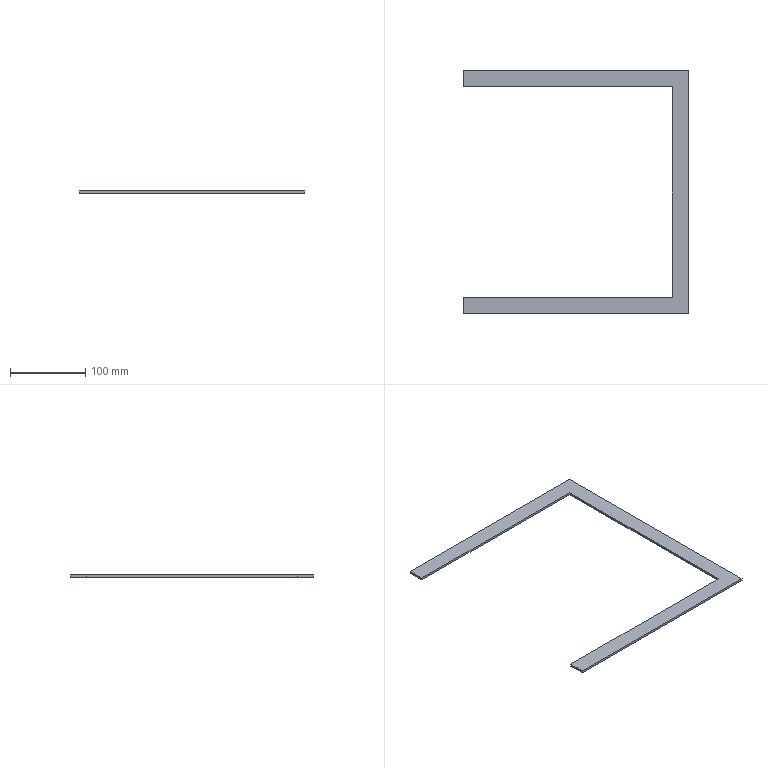Component | SolidWorks | Cover1-9XG1-1 | 1 solid | 10 faces | box 300 x 324 x 3 mm | volume 58080 mm3 | plane 10
build123d program:
from build123d import *

# Parameters (mm, degrees)
BOSS_EXTRUDE1_DEPTH = 3


with BuildPart() as part:
    # Sketch1 → Boss-Extrude1 (new body)
    with BuildSketch(Plane.XY):
        Polygon((-162, 0), (162, 0), (162, 300), (140, 300), (140, 22), (-140, 22), (-140, 300), (-162, 300), align=None)
    extrude(amount=BOSS_EXTRUDE1_DEPTH)


solid = part.part

# Placed as in the assembly
solid = solid.moved(Location((150, 0, -3), (0, 0, 90)))
STEP:
#1=CARTESIAN_POINT('',(-5.906,-6.378,-0.1181));
#2=VERTEX_POINT('',#1);
#3=CARTESIAN_POINT('',(5.906,-6.378,-0.1181));
#4=VERTEX_POINT('',#3);
#5=CARTESIAN_POINT('',(-5.906,-6.378,-0.1181));
#6=DIRECTION('',(1.,0.,-0.));
#7=VECTOR('',#6,39.37);
#8=LINE('',#5,#7);
#9=EDGE_CURVE('',#2,#4,#8,.T.);
#10=ORIENTED_EDGE('',*,*,#9,.T.);
#11=CARTESIAN_POINT('',(5.906,-6.378,-0.));
#12=VERTEX_POINT('',#11);
#13=CARTESIAN_POINT('',(5.906,-6.378,-0.));
#14=DIRECTION('',(0.,-0.,-1.));
#15=VECTOR('',#14,39.37);
#16=LINE('',#13,#15);
#17=EDGE_CURVE('',#12,#4,#16,.T.);
#18=ORIENTED_EDGE('',*,*,#17,.F.);
#19=CARTESIAN_POINT('',(-5.906,-6.378,-0.));
#20=VERTEX_POINT('',#19);
#21=CARTESIAN_POINT('',(-5.906,-6.378,-0.));
#22=DIRECTION('',(1.,0.,-0.));
#23=VECTOR('',#22,39.37);
#24=LINE('',#21,#23);
#25=EDGE_CURVE('',#20,#12,#24,.T.);
#26=ORIENTED_EDGE('',*,*,#25,.F.);
#27=CARTESIAN_POINT('',(-5.906,-6.378,-0.));
#28=DIRECTION('',(0.,-0.,-1.));
#29=VECTOR('',#28,39.37);
#30=LINE('',#27,#29);
#31=EDGE_CURVE('',#20,#2,#30,.T.);
#32=ORIENTED_EDGE('',*,*,#31,.T.);
#33=EDGE_LOOP('',(#10,#18,#26,#32));
#34=FACE_OUTER_BOUND('',#33,.T.);
#35=CARTESIAN_POINT('',(-5.906,-6.378,-0.));
#36=DIRECTION('',(-0.,1.,-0.));
#37=DIRECTION('',(-1.,-0.,0.));
#38=AXIS2_PLACEMENT_3D('',#35,#36,#37);
#39=PLANE('',#38);
#40=ADVANCED_FACE('',(#34),#39,.F.);
#41=CARTESIAN_POINT('',(5.906,6.378,-0.1181));
#42=VERTEX_POINT('',#41);
#43=CARTESIAN_POINT('',(5.906,-6.378,-0.1181));
#44=DIRECTION('',(0.,1.,-0.));
#45=VECTOR('',#44,39.37);
#46=LINE('',#43,#45);
#47=EDGE_CURVE('',#4,#42,#46,.T.);
#48=ORIENTED_EDGE('',*,*,#47,.T.);
#49=CARTESIAN_POINT('',(5.906,6.378,-0.));
#50=VERTEX_POINT('',#49);
#51=CARTESIAN_POINT('',(5.906,6.378,-0.));
#52=DIRECTION('',(0.,-0.,-1.));
#53=VECTOR('',#52,39.37);
#54=LINE('',#51,#53);
#55=EDGE_CURVE('',#50,#42,#54,.T.);
#56=ORIENTED_EDGE('',*,*,#55,.F.);
#57=CARTESIAN_POINT('',(5.906,-6.378,-0.));
#58=DIRECTION('',(0.,1.,-0.));
#59=VECTOR('',#58,39.37);
#60=LINE('',#57,#59);
#61=EDGE_CURVE('',#12,#50,#60,.T.);
#62=ORIENTED_EDGE('',*,*,#61,.F.);
#63=ORIENTED_EDGE('',*,*,#17,.T.);
#64=EDGE_LOOP('',(#48,#56,#62,#63));
#65=FACE_OUTER_BOUND('',#64,.T.);
#66=CARTESIAN_POINT('',(5.906,-6.378,-0.));
#67=DIRECTION('',(-1.,0.,-0.));
#68=DIRECTION('',(0.,0.,1.));
#69=AXIS2_PLACEMENT_3D('',#66,#67,#68);
#70=PLANE('',#69);
#71=ADVANCED_FACE('',(#65),#70,.F.);
#72=CARTESIAN_POINT('',(-5.906,6.378,-0.1181));
#73=VERTEX_POINT('',#72);
#74=CARTESIAN_POINT('',(5.906,6.378,-0.1181));
#75=DIRECTION('',(-1.,0.,-0.));
#76=VECTOR('',#75,39.37);
#77=LINE('',#74,#76);
#78=EDGE_CURVE('',#42,#73,#77,.T.);
#79=ORIENTED_EDGE('',*,*,#78,.T.);
#80=CARTESIAN_POINT('',(-5.906,6.378,-0.));
#81=VERTEX_POINT('',#80);
#82=CARTESIAN_POINT('',(-5.906,6.378,-0.));
#83=DIRECTION('',(0.,-0.,-1.));
#84=VECTOR('',#83,39.37);
#85=LINE('',#82,#84);
#86=EDGE_CURVE('',#81,#73,#85,.T.);
#87=ORIENTED_EDGE('',*,*,#86,.F.);
#88=CARTESIAN_POINT('',(5.906,6.378,-0.));
#89=DIRECTION('',(-1.,0.,-0.));
#90=VECTOR('',#89,39.37);
#91=LINE('',#88,#90);
#92=EDGE_CURVE('',#50,#81,#91,.T.);
#93=ORIENTED_EDGE('',*,*,#92,.F.);
#94=ORIENTED_EDGE('',*,*,#55,.T.);
#95=EDGE_LOOP('',(#79,#87,#93,#94));
#96=FACE_OUTER_BOUND('',#95,.T.);
#97=CARTESIAN_POINT('',(5.906,6.378,-0.));
#98=DIRECTION('',(-0.,-1.,0.));
#99=DIRECTION('',(1.,-0.,0.));
#100=AXIS2_PLACEMENT_3D('',#97,#98,#99);
#101=PLANE('',#100);
#102=ADVANCED_FACE('',(#96),#101,.F.);
#103=CARTESIAN_POINT('',(-5.906,5.512,-0.1181));
#104=VERTEX_POINT('',#103);
#105=CARTESIAN_POINT('',(-5.906,6.378,-0.1181));
#106=DIRECTION('',(-0.,-1.,0.));
#107=VECTOR('',#106,39.37);
#108=LINE('',#105,#107);
#109=EDGE_CURVE('',#73,#104,#108,.T.);
#110=ORIENTED_EDGE('',*,*,#109,.T.);
#111=CARTESIAN_POINT('',(-5.906,5.512,-0.));
#112=VERTEX_POINT('',#111);
#113=CARTESIAN_POINT('',(-5.906,5.512,-0.));
#114=DIRECTION('',(0.,-0.,-1.));
#115=VECTOR('',#114,39.37);
#116=LINE('',#113,#115);
#117=EDGE_CURVE('',#112,#104,#116,.T.);
#118=ORIENTED_EDGE('',*,*,#117,.F.);
#119=CARTESIAN_POINT('',(-5.906,6.378,-0.));
#120=DIRECTION('',(-0.,-1.,0.));
#121=VECTOR('',#120,39.37);
#122=LINE('',#119,#121);
#123=EDGE_CURVE('',#81,#112,#122,.T.);
#124=ORIENTED_EDGE('',*,*,#123,.F.);
#125=ORIENTED_EDGE('',*,*,#86,.T.);
#126=EDGE_LOOP('',(#110,#118,#124,#125));
#127=FACE_OUTER_BOUND('',#126,.T.);
#128=CARTESIAN_POINT('',(-5.906,6.378,-0.));
#129=DIRECTION('',(1.,-0.,0.));
#130=DIRECTION('',(0.,1.,-0.));
#131=AXIS2_PLACEMENT_3D('',#128,#129,#130);
#132=PLANE('',#131);
#133=ADVANCED_FACE('',(#127),#132,.F.);
#134=CARTESIAN_POINT('',(5.039,5.512,-0.1181));
#135=VERTEX_POINT('',#134);
#136=CARTESIAN_POINT('',(-5.906,5.512,-0.1181));
#137=DIRECTION('',(1.,0.,-0.));
#138=VECTOR('',#137,39.37);
#139=LINE('',#136,#138);
#140=EDGE_CURVE('',#104,#135,#139,.T.);
#141=ORIENTED_EDGE('',*,*,#140,.T.);
#142=CARTESIAN_POINT('',(5.039,5.512,-0.));
#143=VERTEX_POINT('',#142);
#144=CARTESIAN_POINT('',(5.039,5.512,-0.));
#145=DIRECTION('',(0.,-0.,-1.));
#146=VECTOR('',#145,39.37);
#147=LINE('',#144,#146);
#148=EDGE_CURVE('',#143,#135,#147,.T.);
#149=ORIENTED_EDGE('',*,*,#148,.F.);
#150=CARTESIAN_POINT('',(-5.906,5.512,-0.));
#151=DIRECTION('',(1.,0.,-0.));
#152=VECTOR('',#151,39.37);
#153=LINE('',#150,#152);
#154=EDGE_CURVE('',#112,#143,#153,.T.);
#155=ORIENTED_EDGE('',*,*,#154,.F.);
#156=ORIENTED_EDGE('',*,*,#117,.T.);
#157=EDGE_LOOP('',(#141,#149,#155,#156));
#158=FACE_OUTER_BOUND('',#157,.T.);
#159=CARTESIAN_POINT('',(-5.906,5.512,-0.));
#160=DIRECTION('',(-0.,1.,-0.));
#161=DIRECTION('',(-1.,-0.,0.));
#162=AXIS2_PLACEMENT_3D('',#159,#160,#161);
#163=PLANE('',#162);
#164=ADVANCED_FACE('',(#158),#163,.F.);
#165=CARTESIAN_POINT('',(5.039,-5.512,-0.1181));
#166=VERTEX_POINT('',#165);
#167=CARTESIAN_POINT('',(5.039,5.512,-0.1181));
#168=DIRECTION('',(0.,-1.,0.));
#169=VECTOR('',#168,39.37);
#170=LINE('',#167,#169);
#171=EDGE_CURVE('',#135,#166,#170,.T.);
#172=ORIENTED_EDGE('',*,*,#171,.T.);
#173=CARTESIAN_POINT('',(5.039,-5.512,-0.));
#174=VERTEX_POINT('',#173);
#175=CARTESIAN_POINT('',(5.039,-5.512,-0.));
#176=DIRECTION('',(0.,-0.,-1.));
#177=VECTOR('',#176,39.37);
#178=LINE('',#175,#177);
#179=EDGE_CURVE('',#174,#166,#178,.T.);
#180=ORIENTED_EDGE('',*,*,#179,.F.);
#181=CARTESIAN_POINT('',(5.039,5.512,-0.));
#182=DIRECTION('',(0.,-1.,0.));
#183=VECTOR('',#182,39.37);
#184=LINE('',#181,#183);
#185=EDGE_CURVE('',#143,#174,#184,.T.);
#186=ORIENTED_EDGE('',*,*,#185,.F.);
#187=ORIENTED_EDGE('',*,*,#148,.T.);
#188=EDGE_LOOP('',(#172,#180,#186,#187));
#189=FACE_OUTER_BOUND('',#188,.T.);
#190=CARTESIAN_POINT('',(5.039,5.512,-0.));
#191=DIRECTION('',(1.,0.,-0.));
#192=DIRECTION('',(-0.,1.,-0.));
#193=AXIS2_PLACEMENT_3D('',#190,#191,#192);
#194=PLANE('',#193);
#195=ADVANCED_FACE('',(#189),#194,.F.);
#196=CARTESIAN_POINT('',(-5.906,-5.512,-0.1181));
#197=VERTEX_POINT('',#196);
#198=CARTESIAN_POINT('',(5.039,-5.512,-0.1181));
#199=DIRECTION('',(-1.,0.,0.));
#200=VECTOR('',#199,39.37);
#201=LINE('',#198,#200);
#202=EDGE_CURVE('',#166,#197,#201,.T.);
#203=ORIENTED_EDGE('',*,*,#202,.T.);
#204=CARTESIAN_POINT('',(-5.906,-5.512,-0.));
#205=VERTEX_POINT('',#204);
#206=CARTESIAN_POINT('',(-5.906,-5.512,-0.));
#207=DIRECTION('',(0.,-0.,-1.));
#208=VECTOR('',#207,39.37);
#209=LINE('',#206,#208);
#210=EDGE_CURVE('',#205,#197,#209,.T.);
#211=ORIENTED_EDGE('',*,*,#210,.F.);
#212=CARTESIAN_POINT('',(5.039,-5.512,-0.));
#213=DIRECTION('',(-1.,0.,0.));
#214=VECTOR('',#213,39.37);
#215=LINE('',#212,#214);
#216=EDGE_CURVE('',#174,#205,#215,.T.);
#217=ORIENTED_EDGE('',*,*,#216,.F.);
#218=ORIENTED_EDGE('',*,*,#179,.T.);
#219=EDGE_LOOP('',(#203,#211,#217,#218));
#220=FACE_OUTER_BOUND('',#219,.T.);
#221=CARTESIAN_POINT('',(5.039,-5.512,-0.));
#222=DIRECTION('',(-0.,-1.,0.));
#223=DIRECTION('',(0.,0.,1.));
#224=AXIS2_PLACEMENT_3D('',#221,#222,#223);
#225=PLANE('',#224);
#226=ADVANCED_FACE('',(#220),#225,.F.);
#227=CARTESIAN_POINT('',(-5.906,-5.512,-0.1181));
#228=DIRECTION('',(-0.,-1.,0.));
#229=VECTOR('',#228,39.37);
#230=LINE('',#227,#229);
#231=EDGE_CURVE('',#197,#2,#230,.T.);
#232=ORIENTED_EDGE('',*,*,#231,.T.);
#233=ORIENTED_EDGE('',*,*,#31,.F.);
#234=CARTESIAN_POINT('',(-5.906,-5.512,-0.));
#235=DIRECTION('',(-0.,-1.,0.));
#236=VECTOR('',#235,39.37);
#237=LINE('',#234,#236);
#238=EDGE_CURVE('',#205,#20,#237,.T.);
#239=ORIENTED_EDGE('',*,*,#238,.F.);
#240=ORIENTED_EDGE('',*,*,#210,.T.);
#241=EDGE_LOOP('',(#232,#233,#239,#240));
#242=FACE_OUTER_BOUND('',#241,.T.);
#243=CARTESIAN_POINT('',(-5.906,-5.512,-0.));
#244=DIRECTION('',(1.,-0.,0.));
#245=DIRECTION('',(0.,-0.,-1.));
#246=AXIS2_PLACEMENT_3D('',#243,#244,#245);
#247=PLANE('',#246);
#248=ADVANCED_FACE('',(#242),#247,.F.);
#249=ORIENTED_EDGE('',*,*,#25,.T.);
#250=ORIENTED_EDGE('',*,*,#61,.T.);
#251=ORIENTED_EDGE('',*,*,#92,.T.);
#252=ORIENTED_EDGE('',*,*,#123,.T.);
#253=ORIENTED_EDGE('',*,*,#154,.T.);
#254=ORIENTED_EDGE('',*,*,#185,.T.);
#255=ORIENTED_EDGE('',*,*,#216,.T.);
#256=ORIENTED_EDGE('',*,*,#238,.T.);
#257=EDGE_LOOP('',(#249,#250,#251,#252,#253,#254,#255,#256));
#258=FACE_OUTER_BOUND('',#257,.T.);
#259=CARTESIAN_POINT('',(5.906,-0.,-0.));
#260=DIRECTION('',(0.,0.,1.));
#261=DIRECTION('',(0.,1.,-0.));
#262=AXIS2_PLACEMENT_3D('',#259,#260,#261);
#263=PLANE('',#262);
#264=ADVANCED_FACE('',(#258),#263,.T.);
#265=ORIENTED_EDGE('',*,*,#9,.F.);
#266=ORIENTED_EDGE('',*,*,#231,.F.);
#267=ORIENTED_EDGE('',*,*,#202,.F.);
#268=ORIENTED_EDGE('',*,*,#171,.F.);
#269=ORIENTED_EDGE('',*,*,#140,.F.);
#270=ORIENTED_EDGE('',*,*,#109,.F.);
#271=ORIENTED_EDGE('',*,*,#78,.F.);
#272=ORIENTED_EDGE('',*,*,#47,.F.);
#273=EDGE_LOOP('',(#265,#266,#267,#268,#269,#270,#271,#272));
#274=FACE_OUTER_BOUND('',#273,.T.);
#275=CARTESIAN_POINT('',(5.906,-0.,-0.1181));
#276=DIRECTION('',(0.,0.,1.));
#277=DIRECTION('',(0.,1.,-0.));
#278=AXIS2_PLACEMENT_3D('',#275,#276,#277);
#279=PLANE('',#278);
#280=ADVANCED_FACE('',(#274),#279,.F.);
#281=CLOSED_SHELL('',(#40,#71,#102,#133,#164,#195,#226,#248,#264,#280));
#282=MANIFOLD_SOLID_BREP('',#281);
#283=CARTESIAN_POINT('',(0.,0.,0.));
#284=DIRECTION('',(0.,0.,1.));
#285=DIRECTION('',(1.,0.,0.));
#286=AXIS2_PLACEMENT_3D('',#283,#284,#285);
#287=(LENGTH_UNIT()NAMED_UNIT(*)SI_UNIT($,.METRE.));
#288=LENGTH_MEASURE_WITH_UNIT(LENGTH_MEASURE(0.0254),#287);
#289=DIMENSIONAL_EXPONENTS(1.,0.,0.,0.,0.,0.,0.);
#290=(CONVERSION_BASED_UNIT('',#288)LENGTH_UNIT()NAMED_UNIT(#289));
#291=UNCERTAINTY_MEASURE_WITH_UNIT(LENGTH_MEASURE(0.00001),#290,'','');
#292=(NAMED_UNIT(*)PLANE_ANGLE_UNIT()SI_UNIT($,.RADIAN.));
#293=(NAMED_UNIT(*)SI_UNIT($,.STERADIAN.)SOLID_ANGLE_UNIT());
#294=(GEOMETRIC_REPRESENTATION_CONTEXT(3)GLOBAL_UNCERTAINTY_ASSIGNED_CONTEXT((#291))GLOBAL_UNIT_ASSIGNED_CONTEXT((#290,#292,#293))REPRESENTATION_CONTEXT('',''));
#295=ADVANCED_BREP_SHAPE_REPRESENTATION('',(#282,#286),#294);
#296=COLOUR_RGB('',0.7922,0.8196,0.9333);
#297=FILL_AREA_STYLE_COLOUR('',#296);
#298=FILL_AREA_STYLE('',(#297));
#299=SURFACE_STYLE_FILL_AREA(#298);
#300=SURFACE_SIDE_STYLE('',(#299));
#301=SURFACE_STYLE_USAGE(.BOTH.,#300);
#302=PRESENTATION_STYLE_ASSIGNMENT((#301));
#303=STYLED_ITEM('',(#302),#282);
#304=PRESENTATION_LAYER_ASSIGNMENT('','',(#303));
#305=(LENGTH_UNIT()NAMED_UNIT(*)SI_UNIT($,.METRE.));
#306=LENGTH_MEASURE_WITH_UNIT(LENGTH_MEASURE(0.0254),#305);
#307=DIMENSIONAL_EXPONENTS(1.,0.,0.,0.,0.,0.,0.);
#308=(CONVERSION_BASED_UNIT('',#306)LENGTH_UNIT()NAMED_UNIT(#307));
#309=UNCERTAINTY_MEASURE_WITH_UNIT(LENGTH_MEASURE(0.00001),#308,'','');
#310=(NAMED_UNIT(*)PLANE_ANGLE_UNIT()SI_UNIT($,.RADIAN.));
#311=(NAMED_UNIT(*)SI_UNIT($,.STERADIAN.)SOLID_ANGLE_UNIT());
#312=(GEOMETRIC_REPRESENTATION_CONTEXT(3)GLOBAL_UNCERTAINTY_ASSIGNED_CONTEXT((#309))GLOBAL_UNIT_ASSIGNED_CONTEXT((#308,#310,#311))REPRESENTATION_CONTEXT('',''));
#313=MECHANICAL_DESIGN_GEOMETRIC_PRESENTATION_REPRESENTATION('',(#303),#312);